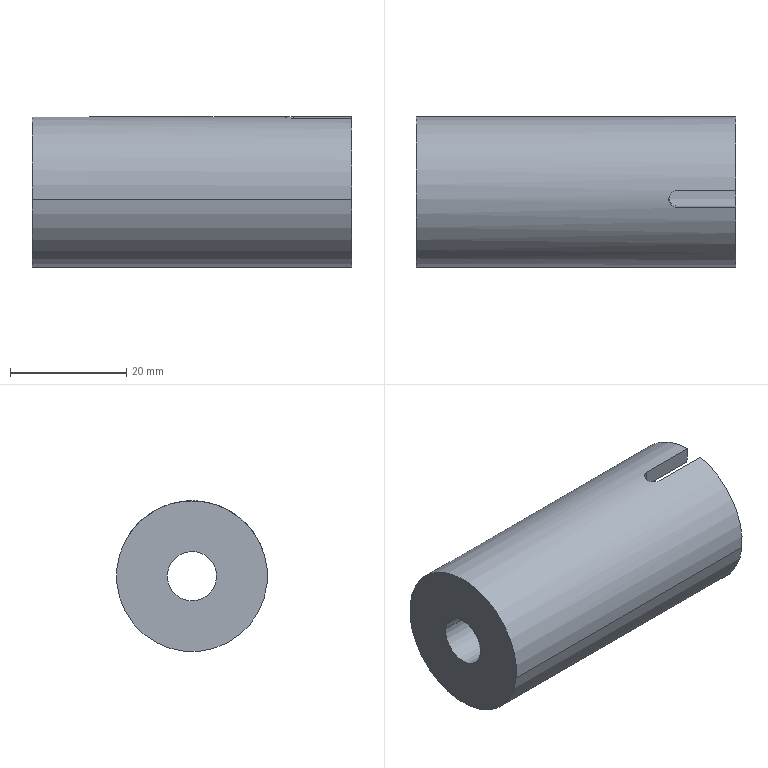Component | SolidWorks | 11HandleSleeve-1 | 1 solid | 15 faces | box 55 x 26 x 26 mm | volume 13302 mm3 | cylinder 9 | plane 6 | commonest cylinder face diameters 8.5 x2 21 x2 20 x2 26 x2 3 x1
build123d program:
from build123d import *

# Parameters (mm, degrees)
SKETCH1_R           = 13
BOSS_EXTRUDE1_DEPTH = 55
SKETCH2_R           = 10
CUT_EXTRUDE1_DEPTH  = 47
SKETCH3_R           = 10.5
CUT_EXTRUDE2_DEPTH  = 2
SKETCH4_R           = 4.25
CUT_EXTRUDE3_DEPTH  = 50
CUT_EXTRUDE4_DEPTH  = 58.991


with BuildPart() as part:
    # Sketch1 → Boss-Extrude1 (new body)
    with BuildSketch(Plane.XY):
        Circle(SKETCH1_R)
    extrude(amount=BOSS_EXTRUDE1_DEPTH)

    # Sketch2 → Cut-Extrude1 (cut)
    with BuildSketch(Plane.XY.offset(55)):
        Circle(SKETCH2_R)
    extrude(amount=-CUT_EXTRUDE1_DEPTH, mode=Mode.SUBTRACT)

    # Sketch3 → Cut-Extrude2 (cut)
    with BuildSketch(Plane.XY.offset(8)):
        Circle(SKETCH3_R)
    extrude(amount=-CUT_EXTRUDE2_DEPTH, mode=Mode.SUBTRACT)

    # Sketch4 → Cut-Extrude3 (cut)
    with BuildSketch(Plane(origin=(0, 0, 0), x_dir=(-1, 0, 0), z_dir=(0, 0, -1))):
        Circle(SKETCH4_R)
    extrude(amount=-CUT_EXTRUDE3_DEPTH, mode=Mode.SUBTRACT)

    # Sketch5 → Cut-Extrude4 (cut, through all)
    with BuildSketch(Plane(origin=(0, 0, 0), x_dir=(1, 0, 0), z_dir=(0, 1, 0))):
        with BuildLine():
            Line((-1.5, -55), (-1.5, -45))
            ThreePointArc((-1.5, -45), (0, -43.5), (1.5, -45))
            Line((1.5, -45), (1.5, -55))
            ThreePointArc((1.5, -55), (0, -56.5), (-1.5, -55))
        make_face()
    extrude(amount=-CUT_EXTRUDE4_DEPTH, mode=Mode.SUBTRACT)


solid = part.part

# Placed as in the assembly
solid = solid.moved(Location((-382, 109.982, -1.287), (-84.304, 90, 0)))
STEP:
#1=COLOUR_RGB('',0.7922,0.8196,0.9333);
#2=FILL_AREA_STYLE_COLOUR('',#1);
#3=FILL_AREA_STYLE('',(#2));
#4=SURFACE_STYLE_FILL_AREA(#3);
#5=SURFACE_SIDE_STYLE('',(#4));
#6=SURFACE_STYLE_USAGE(.BOTH.,#5);
#7=PRESENTATION_STYLE_ASSIGNMENT((#6));
#8=CARTESIAN_POINT('',(-14.803,4.496,-0.03408));
#9=VERTEX_POINT('',#8);
#10=CARTESIAN_POINT('',(-14.803,4.163,-0.06729));
#11=VERTEX_POINT('',#10);
#12=CARTESIAN_POINT('',(-14.803,4.33,-0.05068));
#13=DIRECTION('',(1.,0.,0.));
#14=DIRECTION('',(0.,-0.9951,-0.09924));
#15=AXIS2_PLACEMENT_3D('',#12,#13,#14);
#16=CIRCLE('',#15,0.1673);
#17=EDGE_CURVE('',#9,#11,#16,.T.);
#18=ORIENTED_EDGE('',*,*,#17,.T.);
#19=CARTESIAN_POINT('',(-15.039,4.163,-0.06729));
#20=VERTEX_POINT('',#19);
#21=CARTESIAN_POINT('',(-13.071,4.163,-0.06729));
#22=DIRECTION('',(-1.,-0.,-0.));
#23=VECTOR('',#22,39.37);
#24=LINE('',#21,#23);
#25=EDGE_CURVE('',#11,#20,#24,.T.);
#26=ORIENTED_EDGE('',*,*,#25,.T.);
#27=CARTESIAN_POINT('',(-15.039,4.496,-0.03408));
#28=VERTEX_POINT('',#27);
#29=CARTESIAN_POINT('',(-15.039,4.33,-0.05068));
#30=DIRECTION('',(-1.,-0.,-0.));
#31=DIRECTION('',(0.,0.9951,0.09924));
#32=AXIS2_PLACEMENT_3D('',#29,#30,#31);
#33=CIRCLE('',#32,0.1673);
#34=EDGE_CURVE('',#20,#28,#33,.T.);
#35=ORIENTED_EDGE('',*,*,#34,.T.);
#36=CARTESIAN_POINT('',(-13.071,4.496,-0.03408));
#37=DIRECTION('',(-1.,-0.,-0.));
#38=VECTOR('',#37,39.37);
#39=LINE('',#36,#38);
#40=EDGE_CURVE('',#9,#28,#39,.T.);
#41=ORIENTED_EDGE('',*,*,#40,.F.);
#42=EDGE_LOOP('',(#18,#26,#35,#41));
#43=FACE_OUTER_BOUND('',#42,.T.);
#44=CARTESIAN_POINT('',(-13.071,4.33,-0.05068));
#45=DIRECTION('',(-1.,-0.,-0.));
#46=DIRECTION('',(0.,0.9951,0.09924));
#47=AXIS2_PLACEMENT_3D('',#44,#45,#46);
#48=CYLINDRICAL_SURFACE('',#47,0.1673);
#49=ADVANCED_FACE('',(#43),#48,.F.);
#50=CARTESIAN_POINT('',(-14.803,4.741,-0.009656));
#51=VERTEX_POINT('',#50);
#52=CARTESIAN_POINT('',(-14.803,3.919,-0.09171));
#53=VERTEX_POINT('',#52);
#54=CARTESIAN_POINT('',(-14.803,4.33,-0.05068));
#55=DIRECTION('',(1.,0.,0.));
#56=DIRECTION('',(0.,-0.9951,-0.09924));
#57=AXIS2_PLACEMENT_3D('',#54,#55,#56);
#58=CIRCLE('',#57,0.4134);
#59=EDGE_CURVE('',#51,#53,#58,.T.);
#60=ORIENTED_EDGE('',*,*,#59,.F.);
#61=CARTESIAN_POINT('',(-14.724,4.741,-0.009656));
#62=VERTEX_POINT('',#61);
#63=CARTESIAN_POINT('',(-14.803,4.741,-0.009656));
#64=DIRECTION('',(1.,0.,0.));
#65=VECTOR('',#64,39.37);
#66=LINE('',#63,#65);
#67=EDGE_CURVE('',#51,#62,#66,.T.);
#68=ORIENTED_EDGE('',*,*,#67,.T.);
#69=CARTESIAN_POINT('',(-14.724,3.919,-0.09171));
#70=VERTEX_POINT('',#69);
#71=CARTESIAN_POINT('',(-14.724,4.33,-0.05068));
#72=DIRECTION('',(1.,0.,0.));
#73=DIRECTION('',(0.,-0.9951,-0.09924));
#74=AXIS2_PLACEMENT_3D('',#71,#72,#73);
#75=CIRCLE('',#74,0.4134);
#76=EDGE_CURVE('',#62,#70,#75,.T.);
#77=ORIENTED_EDGE('',*,*,#76,.T.);
#78=CARTESIAN_POINT('',(-14.803,3.919,-0.09171));
#79=DIRECTION('',(1.,0.,0.));
#80=VECTOR('',#79,39.37);
#81=LINE('',#78,#80);
#82=EDGE_CURVE('',#53,#70,#81,.T.);
#83=ORIENTED_EDGE('',*,*,#82,.F.);
#84=EDGE_LOOP('',(#60,#68,#77,#83));
#85=FACE_OUTER_BOUND('',#84,.T.);
#86=CARTESIAN_POINT('',(-14.803,4.33,-0.05068));
#87=DIRECTION('',(1.,0.,0.));
#88=DIRECTION('',(0.,-0.9951,-0.09924));
#89=AXIS2_PLACEMENT_3D('',#86,#87,#88);
#90=CYLINDRICAL_SURFACE('',#89,0.4134);
#91=ADVANCED_FACE('',(#85),#90,.F.);
#92=CARTESIAN_POINT('',(-14.724,4.722,-0.01161));
#93=VERTEX_POINT('',#92);
#94=CARTESIAN_POINT('',(-14.724,3.938,-0.08975));
#95=VERTEX_POINT('',#94);
#96=CARTESIAN_POINT('',(-14.724,4.33,-0.05068));
#97=DIRECTION('',(1.,0.,0.));
#98=DIRECTION('',(0.,-0.9951,-0.09924));
#99=AXIS2_PLACEMENT_3D('',#96,#97,#98);
#100=CIRCLE('',#99,0.3937);
#101=EDGE_CURVE('',#93,#95,#100,.T.);
#102=ORIENTED_EDGE('',*,*,#101,.F.);
#103=CARTESIAN_POINT('',(-12.874,4.722,-0.01161));
#104=VERTEX_POINT('',#103);
#105=CARTESIAN_POINT('',(-14.724,4.722,-0.01161));
#106=DIRECTION('',(1.,0.,0.));
#107=VECTOR('',#106,39.37);
#108=LINE('',#105,#107);
#109=EDGE_CURVE('',#93,#104,#108,.T.);
#110=ORIENTED_EDGE('',*,*,#109,.T.);
#111=CARTESIAN_POINT('',(-12.874,4.35,0.3425));
#112=VERTEX_POINT('',#111);
#113=CARTESIAN_POINT('',(-12.874,4.33,-0.05068));
#114=DIRECTION('',(1.,0.,0.));
#115=DIRECTION('',(0.,-0.9951,-0.09924));
#116=AXIS2_PLACEMENT_3D('',#113,#114,#115);
#117=CIRCLE('',#116,0.3937);
#118=EDGE_CURVE('',#104,#112,#117,.T.);
#119=ORIENTED_EDGE('',*,*,#118,.T.);
#120=CARTESIAN_POINT('',(-13.268,4.35,0.3425));
#121=VERTEX_POINT('',#120);
#122=CARTESIAN_POINT('',(-14.724,4.35,0.3425));
#123=DIRECTION('',(-1.,-0.,-0.));
#124=VECTOR('',#123,39.37);
#125=LINE('',#122,#124);
#126=EDGE_CURVE('',#112,#121,#125,.T.);
#127=ORIENTED_EDGE('',*,*,#126,.T.);
#128=CARTESIAN_POINT('',(-13.268,4.233,0.3308));
#129=VERTEX_POINT('',#128);
#130=CARTESIAN_POINT('',(-13.268,4.35,0.3425));
#131=CARTESIAN_POINT('',(-13.272,4.35,0.3425));
#132=CARTESIAN_POINT('',(-13.275,4.35,0.3425));
#133=CARTESIAN_POINT('',(-13.283,4.348,0.3426));
#134=CARTESIAN_POINT('',(-13.287,4.347,0.3427));
#135=CARTESIAN_POINT('',(-13.294,4.344,0.3428));
#136=CARTESIAN_POINT('',(-13.297,4.342,0.3428));
#137=CARTESIAN_POINT('',(-13.304,4.338,0.3429));
#138=CARTESIAN_POINT('',(-13.307,4.335,0.343));
#139=CARTESIAN_POINT('',(-13.315,4.327,0.343));
#140=CARTESIAN_POINT('',(-13.319,4.321,0.343));
#141=CARTESIAN_POINT('',(-13.325,4.306,0.3424));
#142=CARTESIAN_POINT('',(-13.327,4.299,0.3418));
#143=CARTESIAN_POINT('',(-13.327,4.287,0.3407));
#144=CARTESIAN_POINT('',(-13.326,4.283,0.3403));
#145=CARTESIAN_POINT('',(-13.325,4.276,0.3393));
#146=CARTESIAN_POINT('',(-13.324,4.272,0.3388));
#147=CARTESIAN_POINT('',(-13.319,4.261,0.3371));
#148=CARTESIAN_POINT('',(-13.315,4.255,0.3359));
#149=CARTESIAN_POINT('',(-13.307,4.247,0.3342));
#150=CARTESIAN_POINT('',(-13.304,4.244,0.3336));
#151=CARTESIAN_POINT('',(-13.297,4.24,0.3327));
#152=CARTESIAN_POINT('',(-13.294,4.238,0.3322));
#153=CARTESIAN_POINT('',(-13.283,4.234,0.3312));
#154=CARTESIAN_POINT('',(-13.276,4.233,0.3308));
#155=CARTESIAN_POINT('',(-13.268,4.233,0.3308));
#156=B_SPLINE_CURVE_WITH_KNOTS('',3,(#130,#131,#132,#133,#134,#135,#136,#137,#138,#139,#140,#141,#142,#143,#144,#145,#146,#147,#148,#149,#150,#151,#152,#153,#154,#155),.UNSPECIFIED.,.F.,.F.,(4,2,2,2,2,2,2,2,2,2,2,2,4),(0.,0.0002934,0.0005869,0.0008803,0.001174,0.001761,0.002348,0.002641,0.002934,0.003521,0.003815,0.004108,0.004695),.UNSPECIFIED.);
#157=EDGE_CURVE('',#121,#129,#156,.T.);
#158=ORIENTED_EDGE('',*,*,#157,.T.);
#159=CARTESIAN_POINT('',(-12.874,4.233,0.3308));
#160=VERTEX_POINT('',#159);
#161=CARTESIAN_POINT('',(-14.724,4.233,0.3308));
#162=DIRECTION('',(1.,0.,0.));
#163=VECTOR('',#162,39.37);
#164=LINE('',#161,#163);
#165=EDGE_CURVE('',#129,#160,#164,.T.);
#166=ORIENTED_EDGE('',*,*,#165,.T.);
#167=CARTESIAN_POINT('',(-12.874,3.938,-0.08975));
#168=VERTEX_POINT('',#167);
#169=CARTESIAN_POINT('',(-12.874,4.33,-0.05068));
#170=DIRECTION('',(1.,0.,0.));
#171=DIRECTION('',(0.,-0.9951,-0.09924));
#172=AXIS2_PLACEMENT_3D('',#169,#170,#171);
#173=CIRCLE('',#172,0.3937);
#174=EDGE_CURVE('',#160,#168,#173,.T.);
#175=ORIENTED_EDGE('',*,*,#174,.T.);
#176=CARTESIAN_POINT('',(-14.724,3.938,-0.08975));
#177=DIRECTION('',(1.,0.,0.));
#178=VECTOR('',#177,39.37);
#179=LINE('',#176,#178);
#180=EDGE_CURVE('',#95,#168,#179,.T.);
#181=ORIENTED_EDGE('',*,*,#180,.F.);
#182=EDGE_LOOP('',(#102,#110,#119,#127,#158,#166,#175,#181));
#183=FACE_OUTER_BOUND('',#182,.T.);
#184=CARTESIAN_POINT('',(-14.724,4.33,-0.05068));
#185=DIRECTION('',(1.,0.,0.));
#186=DIRECTION('',(0.,-0.9951,-0.09924));
#187=AXIS2_PLACEMENT_3D('',#184,#185,#186);
#188=CYLINDRICAL_SURFACE('',#187,0.3937);
#189=ADVANCED_FACE('',(#183),#188,.F.);
#190=CARTESIAN_POINT('',(-12.874,3.821,-0.1015));
#191=VERTEX_POINT('',#190);
#192=CARTESIAN_POINT('',(-12.874,4.839,0.0001119));
#193=VERTEX_POINT('',#192);
#194=CARTESIAN_POINT('',(-12.874,4.33,-0.05068));
#195=DIRECTION('',(1.,0.,0.));
#196=DIRECTION('',(0.,-0.9951,-0.09924));
#197=AXIS2_PLACEMENT_3D('',#194,#195,#196);
#198=CIRCLE('',#197,0.5118);
#199=EDGE_CURVE('',#191,#193,#198,.T.);
#200=ORIENTED_EDGE('',*,*,#199,.F.);
#201=CARTESIAN_POINT('',(-15.039,3.821,-0.1015));
#202=VERTEX_POINT('',#201);
#203=CARTESIAN_POINT('',(-12.874,3.821,-0.1015));
#204=DIRECTION('',(-1.,-0.,-0.));
#205=VECTOR('',#204,39.37);
#206=LINE('',#203,#205);
#207=EDGE_CURVE('',#191,#202,#206,.T.);
#208=ORIENTED_EDGE('',*,*,#207,.T.);
#209=CARTESIAN_POINT('',(-15.039,4.839,0.0001119));
#210=VERTEX_POINT('',#209);
#211=CARTESIAN_POINT('',(-15.039,4.33,-0.05068));
#212=DIRECTION('',(1.,0.,0.));
#213=DIRECTION('',(0.,-0.9951,-0.09924));
#214=AXIS2_PLACEMENT_3D('',#211,#212,#213);
#215=CIRCLE('',#214,0.5118);
#216=EDGE_CURVE('',#202,#210,#215,.T.);
#217=ORIENTED_EDGE('',*,*,#216,.T.);
#218=CARTESIAN_POINT('',(-12.874,4.839,0.0001119));
#219=DIRECTION('',(-1.,-0.,-0.));
#220=VECTOR('',#219,39.37);
#221=LINE('',#218,#220);
#222=EDGE_CURVE('',#193,#210,#221,.T.);
#223=ORIENTED_EDGE('',*,*,#222,.F.);
#224=EDGE_LOOP('',(#200,#208,#217,#223));
#225=FACE_OUTER_BOUND('',#224,.T.);
#226=CARTESIAN_POINT('',(-12.874,4.33,-0.05068));
#227=DIRECTION('',(-1.,-0.,-0.));
#228=DIRECTION('',(0.,0.9951,0.09924));
#229=AXIS2_PLACEMENT_3D('',#226,#227,#228);
#230=CYLINDRICAL_SURFACE('',#229,0.5118);
#231=ADVANCED_FACE('',(#225),#230,.T.);
#232=ORIENTED_EDGE('',*,*,#207,.F.);
#233=CARTESIAN_POINT('',(-12.874,4.221,0.4493));
#234=VERTEX_POINT('',#233);
#235=CARTESIAN_POINT('',(-12.874,4.33,-0.05068));
#236=DIRECTION('',(1.,0.,0.));
#237=DIRECTION('',(0.,-0.9951,-0.09924));
#238=AXIS2_PLACEMENT_3D('',#235,#236,#237);
#239=CIRCLE('',#238,0.5118);
#240=EDGE_CURVE('',#234,#191,#239,.T.);
#241=ORIENTED_EDGE('',*,*,#240,.F.);
#242=CARTESIAN_POINT('',(-13.268,4.221,0.4493));
#243=VERTEX_POINT('',#242);
#244=CARTESIAN_POINT('',(-12.874,4.221,0.4493));
#245=DIRECTION('',(-1.,-0.,-0.));
#246=VECTOR('',#245,39.37);
#247=LINE('',#244,#246);
#248=EDGE_CURVE('',#234,#243,#247,.T.);
#249=ORIENTED_EDGE('',*,*,#248,.T.);
#250=CARTESIAN_POINT('',(-13.268,4.338,0.4611));
#251=VERTEX_POINT('',#250);
#252=CARTESIAN_POINT('',(-13.268,4.221,0.4493));
#253=CARTESIAN_POINT('',(-13.272,4.221,0.4493));
#254=CARTESIAN_POINT('',(-13.275,4.221,0.4494));
#255=CARTESIAN_POINT('',(-13.283,4.223,0.4497));
#256=CARTESIAN_POINT('',(-13.287,4.224,0.45));
#257=CARTESIAN_POINT('',(-13.294,4.227,0.4506));
#258=CARTESIAN_POINT('',(-13.297,4.228,0.451));
#259=CARTESIAN_POINT('',(-13.304,4.233,0.4518));
#260=CARTESIAN_POINT('',(-13.307,4.235,0.4523));
#261=CARTESIAN_POINT('',(-13.315,4.243,0.4537));
#262=CARTESIAN_POINT('',(-13.319,4.25,0.4548));
#263=CARTESIAN_POINT('',(-13.325,4.264,0.4569));
#264=CARTESIAN_POINT('',(-13.327,4.271,0.4578));
#265=CARTESIAN_POINT('',(-13.327,4.283,0.459));
#266=CARTESIAN_POINT('',(-13.326,4.287,0.4593));
#267=CARTESIAN_POINT('',(-13.325,4.294,0.4599));
#268=CARTESIAN_POINT('',(-13.324,4.298,0.4601));
#269=CARTESIAN_POINT('',(-13.321,4.305,0.4605));
#270=CARTESIAN_POINT('',(-13.319,4.309,0.4607));
#271=CARTESIAN_POINT('',(-13.315,4.315,0.4609));
#272=CARTESIAN_POINT('',(-13.312,4.318,0.461));
#273=CARTESIAN_POINT('',(-13.307,4.324,0.4611));
#274=CARTESIAN_POINT('',(-13.304,4.326,0.4611));
#275=CARTESIAN_POINT('',(-13.297,4.33,0.4611));
#276=CARTESIAN_POINT('',(-13.294,4.332,0.4611));
#277=CARTESIAN_POINT('',(-13.283,4.337,0.4611));
#278=CARTESIAN_POINT('',(-13.276,4.338,0.4611));
#279=CARTESIAN_POINT('',(-13.268,4.338,0.4611));
#280=B_SPLINE_CURVE_WITH_KNOTS('',3,(#252,#253,#254,#255,#256,#257,#258,#259,#260,#261,#262,#263,#264,#265,#266,#267,#268,#269,#270,#271,#272,#273,#274,#275,#276,#277,#278,#279),.UNSPECIFIED.,.F.,.F.,(4,2,2,2,2,2,2,2,2,2,2,2,2,4),(0.,0.0002933,0.0005866,0.0008798,0.001173,0.00176,0.002346,0.00264,0.002933,0.003226,0.003519,0.003813,0.004106,0.004693),.UNSPECIFIED.);
#281=EDGE_CURVE('',#243,#251,#280,.T.);
#282=ORIENTED_EDGE('',*,*,#281,.T.);
#283=CARTESIAN_POINT('',(-12.874,4.338,0.4611));
#284=VERTEX_POINT('',#283);
#285=CARTESIAN_POINT('',(-12.874,4.338,0.4611));
#286=DIRECTION('',(1.,0.,0.));
#287=VECTOR('',#286,39.37);
#288=LINE('',#285,#287);
#289=EDGE_CURVE('',#251,#284,#288,.T.);
#290=ORIENTED_EDGE('',*,*,#289,.T.);
#291=CARTESIAN_POINT('',(-12.874,4.33,-0.05068));
#292=DIRECTION('',(1.,0.,0.));
#293=DIRECTION('',(0.,-0.9951,-0.09924));
#294=AXIS2_PLACEMENT_3D('',#291,#292,#293);
#295=CIRCLE('',#294,0.5118);
#296=EDGE_CURVE('',#193,#284,#295,.T.);
#297=ORIENTED_EDGE('',*,*,#296,.F.);
#298=ORIENTED_EDGE('',*,*,#222,.T.);
#299=CARTESIAN_POINT('',(-15.039,4.33,-0.05068));
#300=DIRECTION('',(1.,0.,0.));
#301=DIRECTION('',(0.,-0.9951,-0.09924));
#302=AXIS2_PLACEMENT_3D('',#299,#300,#301);
#303=CIRCLE('',#302,0.5118);
#304=EDGE_CURVE('',#210,#202,#303,.T.);
#305=ORIENTED_EDGE('',*,*,#304,.T.);
#306=EDGE_LOOP('',(#232,#241,#249,#282,#290,#297,#298,#305));
#307=FACE_OUTER_BOUND('',#306,.T.);
#308=CARTESIAN_POINT('',(-12.874,4.33,-0.05068));
#309=DIRECTION('',(-1.,-0.,-0.));
#310=DIRECTION('',(0.,0.9951,0.09924));
#311=AXIS2_PLACEMENT_3D('',#308,#309,#310);
#312=CYLINDRICAL_SURFACE('',#311,0.5118);
#313=ADVANCED_FACE('',(#307),#312,.T.);
#314=CARTESIAN_POINT('',(-12.874,4.338,0.4645));
#315=DIRECTION('',(0.,0.09924,-0.9951));
#316=VECTOR('',#315,39.37);
#317=LINE('',#314,#316);
#318=EDGE_CURVE('',#284,#112,#317,.T.);
#319=ORIENTED_EDGE('',*,*,#318,.T.);
#320=ORIENTED_EDGE('',*,*,#118,.F.);
#321=CARTESIAN_POINT('',(-12.874,4.33,-0.05068));
#322=DIRECTION('',(1.,0.,0.));
#323=DIRECTION('',(0.,-0.9951,-0.09924));
#324=AXIS2_PLACEMENT_3D('',#321,#322,#323);
#325=CIRCLE('',#324,0.3937);
#326=EDGE_CURVE('',#168,#104,#325,.T.);
#327=ORIENTED_EDGE('',*,*,#326,.F.);
#328=ORIENTED_EDGE('',*,*,#174,.F.);
#329=CARTESIAN_POINT('',(-12.874,4.22,0.4527));
#330=DIRECTION('',(0.,0.09924,-0.9951));
#331=VECTOR('',#330,39.37);
#332=LINE('',#329,#331);
#333=EDGE_CURVE('',#234,#160,#332,.T.);
#334=ORIENTED_EDGE('',*,*,#333,.F.);
#335=ORIENTED_EDGE('',*,*,#240,.T.);
#336=ORIENTED_EDGE('',*,*,#199,.T.);
#337=ORIENTED_EDGE('',*,*,#296,.T.);
#338=EDGE_LOOP('',(#319,#320,#327,#328,#334,#335,#336,#337));
#339=FACE_OUTER_BOUND('',#338,.T.);
#340=CARTESIAN_POINT('',(-12.874,4.33,-0.05068));
#341=DIRECTION('',(1.,0.,0.));
#342=DIRECTION('',(0.,-0.9951,-0.09924));
#343=AXIS2_PLACEMENT_3D('',#340,#341,#342);
#344=PLANE('',#343);
#345=ADVANCED_FACE('',(#339),#344,.T.);
#346=CARTESIAN_POINT('',(-15.039,4.33,-0.05068));
#347=DIRECTION('',(-1.,-0.,-0.));
#348=DIRECTION('',(0.,0.9951,0.09924));
#349=AXIS2_PLACEMENT_3D('',#346,#347,#348);
#350=CIRCLE('',#349,0.1673);
#351=EDGE_CURVE('',#28,#20,#350,.T.);
#352=ORIENTED_EDGE('',*,*,#351,.F.);
#353=ORIENTED_EDGE('',*,*,#34,.F.);
#354=EDGE_LOOP('',(#352,#353));
#355=FACE_BOUND('',#354,.T.);
#356=ORIENTED_EDGE('',*,*,#304,.F.);
#357=ORIENTED_EDGE('',*,*,#216,.F.);
#358=EDGE_LOOP('',(#356,#357));
#359=FACE_OUTER_BOUND('',#358,.T.);
#360=CARTESIAN_POINT('',(-15.039,4.33,-0.05068));
#361=DIRECTION('',(1.,0.,0.));
#362=DIRECTION('',(0.,-0.9951,-0.09924));
#363=AXIS2_PLACEMENT_3D('',#360,#361,#362);
#364=PLANE('',#363);
#365=ADVANCED_FACE('',(#355,#359),#364,.F.);
#366=ORIENTED_EDGE('',*,*,#109,.F.);
#367=CARTESIAN_POINT('',(-14.724,4.33,-0.05068));
#368=DIRECTION('',(1.,0.,0.));
#369=DIRECTION('',(0.,-0.9951,-0.09924));
#370=AXIS2_PLACEMENT_3D('',#367,#368,#369);
#371=CIRCLE('',#370,0.3937);
#372=EDGE_CURVE('',#95,#93,#371,.T.);
#373=ORIENTED_EDGE('',*,*,#372,.F.);
#374=ORIENTED_EDGE('',*,*,#180,.T.);
#375=ORIENTED_EDGE('',*,*,#326,.T.);
#376=EDGE_LOOP('',(#366,#373,#374,#375));
#377=FACE_OUTER_BOUND('',#376,.T.);
#378=CARTESIAN_POINT('',(-14.724,4.33,-0.05068));
#379=DIRECTION('',(1.,0.,0.));
#380=DIRECTION('',(0.,-0.9951,-0.09924));
#381=AXIS2_PLACEMENT_3D('',#378,#379,#380);
#382=CYLINDRICAL_SURFACE('',#381,0.3937);
#383=ADVANCED_FACE('',(#377),#382,.F.);
#384=ORIENTED_EDGE('',*,*,#67,.F.);
#385=CARTESIAN_POINT('',(-14.803,4.33,-0.05068));
#386=DIRECTION('',(1.,0.,0.));
#387=DIRECTION('',(0.,-0.9951,-0.09924));
#388=AXIS2_PLACEMENT_3D('',#385,#386,#387);
#389=CIRCLE('',#388,0.4134);
#390=EDGE_CURVE('',#53,#51,#389,.T.);
#391=ORIENTED_EDGE('',*,*,#390,.F.);
#392=ORIENTED_EDGE('',*,*,#82,.T.);
#393=CARTESIAN_POINT('',(-14.724,4.33,-0.05068));
#394=DIRECTION('',(1.,0.,0.));
#395=DIRECTION('',(0.,-0.9951,-0.09924));
#396=AXIS2_PLACEMENT_3D('',#393,#394,#395);
#397=CIRCLE('',#396,0.4134);
#398=EDGE_CURVE('',#70,#62,#397,.T.);
#399=ORIENTED_EDGE('',*,*,#398,.T.);
#400=EDGE_LOOP('',(#384,#391,#392,#399));
#401=FACE_OUTER_BOUND('',#400,.T.);
#402=CARTESIAN_POINT('',(-14.803,4.33,-0.05068));
#403=DIRECTION('',(1.,0.,0.));
#404=DIRECTION('',(0.,-0.9951,-0.09924));
#405=AXIS2_PLACEMENT_3D('',#402,#403,#404);
#406=CYLINDRICAL_SURFACE('',#405,0.4134);
#407=ADVANCED_FACE('',(#401),#406,.F.);
#408=ORIENTED_EDGE('',*,*,#17,.F.);
#409=CARTESIAN_POINT('',(-14.803,4.33,-0.05068));
#410=DIRECTION('',(1.,0.,0.));
#411=DIRECTION('',(0.,-0.9951,-0.09924));
#412=AXIS2_PLACEMENT_3D('',#409,#410,#411);
#413=CIRCLE('',#412,0.1673);
#414=EDGE_CURVE('',#11,#9,#413,.T.);
#415=ORIENTED_EDGE('',*,*,#414,.F.);
#416=EDGE_LOOP('',(#408,#415));
#417=FACE_BOUND('',#416,.T.);
#418=ORIENTED_EDGE('',*,*,#390,.T.);
#419=ORIENTED_EDGE('',*,*,#59,.T.);
#420=EDGE_LOOP('',(#418,#419));
#421=FACE_OUTER_BOUND('',#420,.T.);
#422=CARTESIAN_POINT('',(-14.803,4.33,-0.05068));
#423=DIRECTION('',(1.,0.,0.));
#424=DIRECTION('',(0.,-0.9951,-0.09924));
#425=AXIS2_PLACEMENT_3D('',#422,#423,#424);
#426=PLANE('',#425);
#427=ADVANCED_FACE('',(#417,#421),#426,.T.);
#428=ORIENTED_EDGE('',*,*,#372,.T.);
#429=ORIENTED_EDGE('',*,*,#101,.T.);
#430=EDGE_LOOP('',(#428,#429));
#431=FACE_BOUND('',#430,.T.);
#432=ORIENTED_EDGE('',*,*,#398,.F.);
#433=ORIENTED_EDGE('',*,*,#76,.F.);
#434=EDGE_LOOP('',(#432,#433));
#435=FACE_OUTER_BOUND('',#434,.T.);
#436=CARTESIAN_POINT('',(-14.724,4.33,-0.05068));
#437=DIRECTION('',(1.,0.,0.));
#438=DIRECTION('',(0.,-0.9951,-0.09924));
#439=AXIS2_PLACEMENT_3D('',#436,#437,#438);
#440=PLANE('',#439);
#441=ADVANCED_FACE('',(#431,#435),#440,.F.);
#442=ORIENTED_EDGE('',*,*,#25,.F.);
#443=ORIENTED_EDGE('',*,*,#414,.T.);
#444=ORIENTED_EDGE('',*,*,#40,.T.);
#445=ORIENTED_EDGE('',*,*,#351,.T.);
#446=EDGE_LOOP('',(#442,#443,#444,#445));
#447=FACE_OUTER_BOUND('',#446,.T.);
#448=CARTESIAN_POINT('',(-13.071,4.33,-0.05068));
#449=DIRECTION('',(-1.,-0.,-0.));
#450=DIRECTION('',(0.,0.9951,0.09924));
#451=AXIS2_PLACEMENT_3D('',#448,#449,#450);
#452=CYLINDRICAL_SURFACE('',#451,0.1673);
#453=ADVANCED_FACE('',(#447),#452,.F.);
#454=CARTESIAN_POINT('',(-13.268,4.338,0.4645));
#455=DIRECTION('',(0.,0.09924,-0.9951));
#456=VECTOR('',#455,39.37);
#457=LINE('',#454,#456);
#458=EDGE_CURVE('',#251,#121,#457,.T.);
#459=ORIENTED_EDGE('',*,*,#458,.T.);
#460=ORIENTED_EDGE('',*,*,#126,.F.);
#461=ORIENTED_EDGE('',*,*,#318,.F.);
#462=ORIENTED_EDGE('',*,*,#289,.F.);
#463=EDGE_LOOP('',(#459,#460,#461,#462));
#464=FACE_OUTER_BOUND('',#463,.T.);
#465=CARTESIAN_POINT('',(-12.874,4.338,0.4645));
#466=DIRECTION('',(-0.,0.9951,0.09924));
#467=DIRECTION('',(1.,0.,0.));
#468=AXIS2_PLACEMENT_3D('',#465,#466,#467);
#469=PLANE('',#468);
#470=ADVANCED_FACE('',(#464),#469,.F.);
#471=CARTESIAN_POINT('',(-13.268,4.22,0.4527));
#472=DIRECTION('',(0.,0.09924,-0.9951));
#473=VECTOR('',#472,39.37);
#474=LINE('',#471,#473);
#475=EDGE_CURVE('',#243,#129,#474,.T.);
#476=ORIENTED_EDGE('',*,*,#475,.T.);
#477=ORIENTED_EDGE('',*,*,#157,.F.);
#478=ORIENTED_EDGE('',*,*,#458,.F.);
#479=ORIENTED_EDGE('',*,*,#281,.F.);
#480=EDGE_LOOP('',(#476,#477,#478,#479));
#481=FACE_OUTER_BOUND('',#480,.T.);
#482=CARTESIAN_POINT('',(-13.268,4.279,0.4586));
#483=DIRECTION('',(0.,0.09924,-0.9951));
#484=DIRECTION('',(1.,0.,0.));
#485=AXIS2_PLACEMENT_3D('',#482,#483,#484);
#486=CYLINDRICAL_SURFACE('',#485,0.05906);
#487=ADVANCED_FACE('',(#481),#486,.F.);
#488=ORIENTED_EDGE('',*,*,#333,.T.);
#489=ORIENTED_EDGE('',*,*,#165,.F.);
#490=ORIENTED_EDGE('',*,*,#475,.F.);
#491=ORIENTED_EDGE('',*,*,#248,.F.);
#492=EDGE_LOOP('',(#488,#489,#490,#491));
#493=FACE_OUTER_BOUND('',#492,.T.);
#494=CARTESIAN_POINT('',(-12.874,4.22,0.4527));
#495=DIRECTION('',(0.,-0.9951,-0.09924));
#496=DIRECTION('',(-1.,-0.,-0.));
#497=AXIS2_PLACEMENT_3D('',#494,#495,#496);
#498=PLANE('',#497);
#499=ADVANCED_FACE('',(#493),#498,.F.);
#500=CLOSED_SHELL('',(#49,#91,#189,#231,#313,#345,#365,#383,#407,#427,#441,#453,#470,#487,#499));
#501=MANIFOLD_SOLID_BREP('',#500);
#502=STYLED_ITEM('',(#7),#501);
#503=PRESENTATION_LAYER_ASSIGNMENT('','',(#502));
#504=CARTESIAN_POINT('',(0.,0.,0.));
#505=DIRECTION('',(0.,0.,1.));
#506=DIRECTION('',(1.,0.,0.));
#507=AXIS2_PLACEMENT_3D('',#504,#505,#506);
#508=(LENGTH_UNIT()NAMED_UNIT(*)SI_UNIT($,.METRE.));
#509=LENGTH_MEASURE_WITH_UNIT(LENGTH_MEASURE(0.0254),#508);
#510=DIMENSIONAL_EXPONENTS(1.,0.,0.,0.,0.,0.,0.);
#511=(CONVERSION_BASED_UNIT('',#509)LENGTH_UNIT()NAMED_UNIT(#510));
#512=UNCERTAINTY_MEASURE_WITH_UNIT(LENGTH_MEASURE(0.00001),#511,'','');
#513=(NAMED_UNIT(*)PLANE_ANGLE_UNIT()SI_UNIT($,.RADIAN.));
#514=(NAMED_UNIT(*)SI_UNIT($,.STERADIAN.)SOLID_ANGLE_UNIT());
#515=(GEOMETRIC_REPRESENTATION_CONTEXT(3)GLOBAL_UNCERTAINTY_ASSIGNED_CONTEXT((#512))GLOBAL_UNIT_ASSIGNED_CONTEXT((#511,#513,#514))REPRESENTATION_CONTEXT('',''));
#516=ADVANCED_BREP_SHAPE_REPRESENTATION('',(#501,#507),#515);
#517=(LENGTH_UNIT()NAMED_UNIT(*)SI_UNIT($,.METRE.));
#518=LENGTH_MEASURE_WITH_UNIT(LENGTH_MEASURE(0.0254),#517);
#519=DIMENSIONAL_EXPONENTS(1.,0.,0.,0.,0.,0.,0.);
#520=(CONVERSION_BASED_UNIT('',#518)LENGTH_UNIT()NAMED_UNIT(#519));
#521=UNCERTAINTY_MEASURE_WITH_UNIT(LENGTH_MEASURE(0.00001),#520,'','');
#522=(NAMED_UNIT(*)PLANE_ANGLE_UNIT()SI_UNIT($,.RADIAN.));
#523=(NAMED_UNIT(*)SI_UNIT($,.STERADIAN.)SOLID_ANGLE_UNIT());
#524=(GEOMETRIC_REPRESENTATION_CONTEXT(3)GLOBAL_UNCERTAINTY_ASSIGNED_CONTEXT((#521))GLOBAL_UNIT_ASSIGNED_CONTEXT((#520,#522,#523))REPRESENTATION_CONTEXT('',''));
#525=MECHANICAL_DESIGN_GEOMETRIC_PRESENTATION_REPRESENTATION('',(#502),#524);